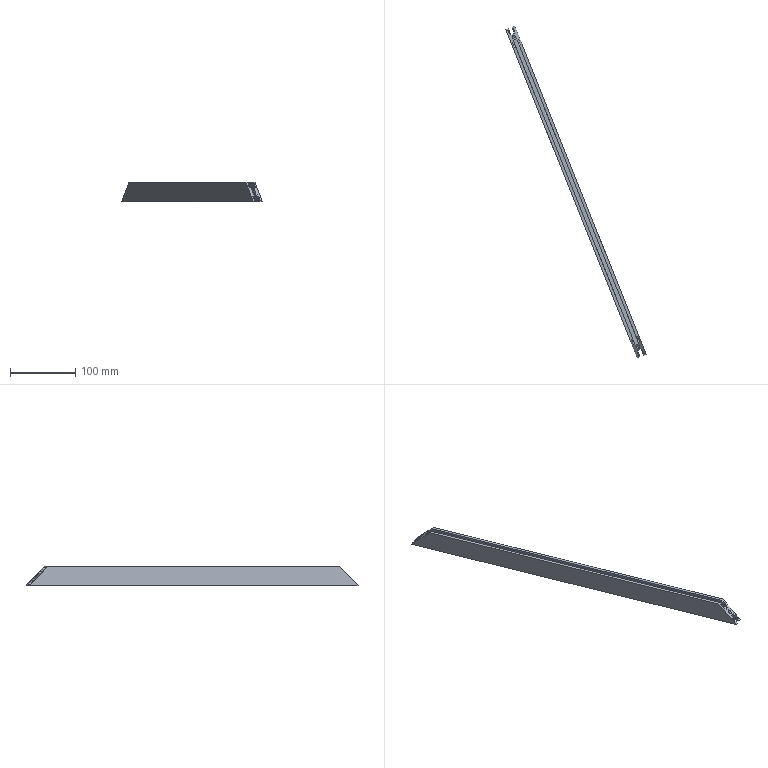Component | SolidWorks | GuardDoor-1_3015-542.5-2 | 1 solid | 32 faces | box 215.79 x 509.13 x 30 mm | volume 130208 mm3 | plane 30 | cylinder 2 | commonest cylinder face diameters 5 x2
build123d program:
from build123d import *

# Parameters (mm, degrees)
SKETCH1_R           = 2.5
BOSS_EXTRUDE1_DEPTH = 542.5
CUT_EXTRUDE1_DEPTH  = 18
CUT_EXTRUDE2_DEPTH  = 18


with BuildPart() as part:
    # Sketch1 → Boss-Extrude1 (new body)
    with BuildSketch(Plane.XY):
        Polygon((0, 0), (30, 0), (30, -4.35), (27.5, -4.35), (27.5, -2.35), (22, -2.35), (22, -4.35), (19.5, -4.35), (19.5, -10.65), (22, -10.65), (22, -12.65), (27.5, -12.65), (27.5, -10.65), (30, -10.65), (30, -15), (0, -15), (0, -10.65), (2.5, -10.65), (2.5, -12.65), (8, -12.65), (8, -10.65), (10.5, -10.65), (10.5, -4.35), (8, -4.35), (8, -2.35), (2.5, -2.35), (2.5, -4.35), (0, -4.35), align=None)
        with Locations((15, -7.5)):
            Circle(SKETCH1_R, mode=Mode.SUBTRACT)
    extrude(amount=BOSS_EXTRUDE1_DEPTH)

    # Sketch2 → Cut-Extrude1 (cut)
    with BuildSketch(Plane(origin=(0, 0, 0), x_dir=(1, 0, 0), z_dir=(0, 1, 0))):
        Polygon((0, 0), (30, -30), (30, 0), align=None)
    extrude(amount=-CUT_EXTRUDE1_DEPTH, mode=Mode.SUBTRACT)

    # Sketch3 → Cut-Extrude2 (cut)
    with BuildSketch(Plane(origin=(0, 0, 0), x_dir=(1, 0, 0), z_dir=(0, 1, 0))):
        Polygon((0, -542.5), (30, -512.5), (30, -542.5), align=None)
    extrude(amount=-CUT_EXTRUDE2_DEPTH, mode=Mode.SUBTRACT)


solid = part.part

# Placed as in the assembly
solid = solid.moved(Location((861.238, 1157.201, -420), (90, 21.845, 90)))
STEP:
#1=COLOUR_RGB('',0.7922,0.8196,0.9333);
#2=FILL_AREA_STYLE_COLOUR('',#1);
#3=FILL_AREA_STYLE('',(#2));
#4=SURFACE_STYLE_FILL_AREA(#3);
#5=SURFACE_SIDE_STYLE('',(#4));
#6=SURFACE_STYLE_USAGE(.BOTH.,#5);
#7=PRESENTATION_STYLE_ASSIGNMENT((#6));
#8=CARTESIAN_POINT('',(41.872,26.484,-15.846));
#9=VERTEX_POINT('',#8);
#10=CARTESIAN_POINT('',(41.945,26.301,-16.043));
#11=VERTEX_POINT('',#10);
#12=CARTESIAN_POINT('',(41.872,26.484,-15.846));
#13=CARTESIAN_POINT('',(42.055,26.557,-15.846));
#14=CARTESIAN_POINT('',(42.128,26.374,-16.043));
#15=CARTESIAN_POINT('',(41.945,26.301,-16.043));
#16=(BOUNDED_CURVE()B_SPLINE_CURVE(3,(#12,#13,#14,#15),.UNSPECIFIED.,.F.,.F.)B_SPLINE_CURVE_WITH_KNOTS((4,4),(-0.,3.142),.UNSPECIFIED.)CURVE()GEOMETRIC_REPRESENTATION_ITEM()RATIONAL_B_SPLINE_CURVE((1.,0.3333,0.3333,1.))REPRESENTATION_ITEM(''));
#17=EDGE_CURVE('',#9,#11,#16,.T.);
#18=ORIENTED_EDGE('',*,*,#17,.F.);
#19=CARTESIAN_POINT('',(34.437,45.029,-15.846));
#20=VERTEX_POINT('',#19);
#21=CARTESIAN_POINT('',(42.129,25.844,-15.846));
#22=DIRECTION('',(-0.3721,0.9282,0.));
#23=VECTOR('',#22,39.37);
#24=LINE('',#21,#23);
#25=EDGE_CURVE('',#9,#20,#24,.T.);
#26=ORIENTED_EDGE('',*,*,#25,.T.);
#27=CARTESIAN_POINT('',(34.364,45.212,-16.043));
#28=VERTEX_POINT('',#27);
#29=CARTESIAN_POINT('',(34.364,45.212,-16.043));
#30=CARTESIAN_POINT('',(34.547,45.285,-16.043));
#31=CARTESIAN_POINT('',(34.62,45.103,-15.846));
#32=CARTESIAN_POINT('',(34.437,45.029,-15.846));
#33=(BOUNDED_CURVE()B_SPLINE_CURVE(3,(#29,#30,#31,#32),.UNSPECIFIED.,.F.,.T.)B_SPLINE_CURVE_WITH_KNOTS((4,4),(-0.,3.142),.UNSPECIFIED.)CURVE()GEOMETRIC_REPRESENTATION_ITEM()RATIONAL_B_SPLINE_CURVE((1.,0.3333,0.3333,1.))REPRESENTATION_ITEM(''));
#34=EDGE_CURVE('',#28,#20,#33,.T.);
#35=ORIENTED_EDGE('',*,*,#34,.F.);
#36=CARTESIAN_POINT('',(42.129,25.844,-16.043));
#37=DIRECTION('',(-0.3721,0.9282,0.));
#38=VECTOR('',#37,39.37);
#39=LINE('',#36,#38);
#40=EDGE_CURVE('',#11,#28,#39,.T.);
#41=ORIENTED_EDGE('',*,*,#40,.F.);
#42=EDGE_LOOP('',(#18,#26,#35,#41));
#43=FACE_OUTER_BOUND('',#42,.T.);
#44=CARTESIAN_POINT('',(42.129,25.844,-15.945));
#45=DIRECTION('',(-0.3721,0.9282,0.));
#46=DIRECTION('',(0.,0.,-1.));
#47=AXIS2_PLACEMENT_3D('',#44,#45,#46);
#48=CYLINDRICAL_SURFACE('',#47,0.09843);
#49=ADVANCED_FACE('',(#43),#48,.F.);
#50=CARTESIAN_POINT('',(33.907,45.559,-16.535));
#51=VERTEX_POINT('',#50);
#52=CARTESIAN_POINT('',(34.066,45.623,-16.535));
#53=VERTEX_POINT('',#52);
#54=CARTESIAN_POINT('',(33.907,45.559,-16.535));
#55=DIRECTION('',(0.9282,0.3721,-0.));
#56=VECTOR('',#55,39.37);
#57=LINE('',#54,#56);
#58=EDGE_CURVE('',#51,#53,#57,.T.);
#59=ORIENTED_EDGE('',*,*,#58,.T.);
#60=CARTESIAN_POINT('',(42.013,25.798,-16.535));
#61=VERTEX_POINT('',#60);
#62=CARTESIAN_POINT('',(42.013,25.798,-16.535));
#63=DIRECTION('',(-0.3721,0.9282,0.));
#64=VECTOR('',#63,39.37);
#65=LINE('',#62,#64);
#66=EDGE_CURVE('',#61,#53,#65,.T.);
#67=ORIENTED_EDGE('',*,*,#66,.F.);
#68=CARTESIAN_POINT('',(41.854,25.735,-16.535));
#69=VERTEX_POINT('',#68);
#70=CARTESIAN_POINT('',(41.854,25.735,-16.535));
#71=DIRECTION('',(0.9282,0.3721,-0.));
#72=VECTOR('',#71,39.37);
#73=LINE('',#70,#72);
#74=EDGE_CURVE('',#69,#61,#73,.T.);
#75=ORIENTED_EDGE('',*,*,#74,.F.);
#76=CARTESIAN_POINT('',(41.854,25.735,-16.535));
#77=DIRECTION('',(-0.3721,0.9282,0.));
#78=VECTOR('',#77,39.37);
#79=LINE('',#76,#78);
#80=EDGE_CURVE('',#69,#51,#79,.T.);
#81=ORIENTED_EDGE('',*,*,#80,.T.);
#82=EDGE_LOOP('',(#59,#67,#75,#81));
#83=FACE_OUTER_BOUND('',#82,.T.);
#84=CARTESIAN_POINT('',(41.854,25.735,-16.535));
#85=DIRECTION('',(0.,-0.,1.));
#86=DIRECTION('',(-0.9282,-0.3721,0.));
#87=AXIS2_PLACEMENT_3D('',#84,#85,#86);
#88=PLANE('',#87);
#89=ADVANCED_FACE('',(#83),#88,.F.);
#90=CARTESIAN_POINT('',(41.977,25.89,-16.437));
#91=VERTEX_POINT('',#90);
#92=CARTESIAN_POINT('',(34.103,45.531,-16.437));
#93=VERTEX_POINT('',#92);
#94=CARTESIAN_POINT('',(42.013,25.798,-16.437));
#95=DIRECTION('',(-0.3721,0.9282,0.));
#96=VECTOR('',#95,39.37);
#97=LINE('',#94,#96);
#98=EDGE_CURVE('',#91,#93,#97,.T.);
#99=ORIENTED_EDGE('',*,*,#98,.F.);
#100=CARTESIAN_POINT('',(42.013,25.798,-16.535));
#101=DIRECTION('',(0.2631,-0.6563,-0.7071));
#102=VECTOR('',#101,39.37);
#103=LINE('',#100,#102);
#104=EDGE_CURVE('',#91,#61,#103,.T.);
#105=ORIENTED_EDGE('',*,*,#104,.T.);
#106=ORIENTED_EDGE('',*,*,#66,.T.);
#107=CARTESIAN_POINT('',(38.04,35.711,-5.856));
#108=DIRECTION('',(0.2631,-0.6563,0.7071));
#109=VECTOR('',#108,39.37);
#110=LINE('',#107,#109);
#111=EDGE_CURVE('',#53,#93,#110,.T.);
#112=ORIENTED_EDGE('',*,*,#111,.T.);
#113=EDGE_LOOP('',(#99,#105,#106,#112));
#114=FACE_OUTER_BOUND('',#113,.T.);
#115=CARTESIAN_POINT('',(42.013,25.798,-16.535));
#116=DIRECTION('',(-0.9282,-0.3721,0.));
#117=DIRECTION('',(0.3721,-0.9282,-0.));
#118=AXIS2_PLACEMENT_3D('',#115,#116,#117);
#119=PLANE('',#118);
#120=ADVANCED_FACE('',(#114),#119,.F.);
#121=CARTESIAN_POINT('',(41.904,25.86,-16.437));
#122=VERTEX_POINT('',#121);
#123=CARTESIAN_POINT('',(34.029,45.502,-16.437));
#124=VERTEX_POINT('',#123);
#125=CARTESIAN_POINT('',(41.94,25.769,-16.437));
#126=DIRECTION('',(-0.3721,0.9282,0.));
#127=VECTOR('',#126,39.37);
#128=LINE('',#125,#127);
#129=EDGE_CURVE('',#122,#124,#128,.T.);
#130=ORIENTED_EDGE('',*,*,#129,.F.);
#131=CARTESIAN_POINT('',(41.977,25.89,-16.437));
#132=DIRECTION('',(0.9282,0.3721,-0.));
#133=VECTOR('',#132,39.37);
#134=LINE('',#131,#133);
#135=EDGE_CURVE('',#122,#91,#134,.T.);
#136=ORIENTED_EDGE('',*,*,#135,.T.);
#137=ORIENTED_EDGE('',*,*,#98,.T.);
#138=CARTESIAN_POINT('',(34.103,45.531,-16.437));
#139=DIRECTION('',(-0.9282,-0.3721,0.));
#140=VECTOR('',#139,39.37);
#141=LINE('',#138,#140);
#142=EDGE_CURVE('',#93,#124,#141,.T.);
#143=ORIENTED_EDGE('',*,*,#142,.T.);
#144=EDGE_LOOP('',(#130,#136,#137,#143));
#145=FACE_OUTER_BOUND('',#144,.T.);
#146=CARTESIAN_POINT('',(42.013,25.798,-16.437));
#147=DIRECTION('',(-0.,0.,-1.));
#148=DIRECTION('',(0.3721,-0.9282,-0.));
#149=AXIS2_PLACEMENT_3D('',#146,#147,#148);
#150=PLANE('',#149);
#151=ADVANCED_FACE('',(#145),#150,.F.);
#152=CARTESIAN_POINT('',(41.823,26.061,-16.22));
#153=VERTEX_POINT('',#152);
#154=CARTESIAN_POINT('',(34.11,45.301,-16.22));
#155=VERTEX_POINT('',#154);
#156=CARTESIAN_POINT('',(41.94,25.769,-16.22));
#157=DIRECTION('',(-0.3721,0.9282,0.));
#158=VECTOR('',#157,39.37);
#159=LINE('',#156,#158);
#160=EDGE_CURVE('',#153,#155,#159,.T.);
#161=ORIENTED_EDGE('',*,*,#160,.F.);
#162=CARTESIAN_POINT('',(41.922,25.815,-16.486));
#163=DIRECTION('',(0.2631,-0.6563,-0.7071));
#164=VECTOR('',#163,39.37);
#165=LINE('',#162,#164);
#166=EDGE_CURVE('',#153,#122,#165,.T.);
#167=ORIENTED_EDGE('',*,*,#166,.T.);
#168=ORIENTED_EDGE('',*,*,#129,.T.);
#169=CARTESIAN_POINT('',(37.985,35.636,-5.807));
#170=DIRECTION('',(0.2631,-0.6563,0.7071));
#171=VECTOR('',#170,39.37);
#172=LINE('',#169,#171);
#173=EDGE_CURVE('',#124,#155,#172,.T.);
#174=ORIENTED_EDGE('',*,*,#173,.T.);
#175=EDGE_LOOP('',(#161,#167,#168,#174));
#176=FACE_OUTER_BOUND('',#175,.T.);
#177=CARTESIAN_POINT('',(41.94,25.769,-16.437));
#178=DIRECTION('',(-0.9282,-0.3721,0.));
#179=DIRECTION('',(0.3721,-0.9282,-0.));
#180=AXIS2_PLACEMENT_3D('',#177,#178,#179);
#181=PLANE('',#180);
#182=ADVANCED_FACE('',(#176),#181,.F.);
#183=CARTESIAN_POINT('',(41.896,26.091,-16.22));
#184=VERTEX_POINT('',#183);
#185=CARTESIAN_POINT('',(34.183,45.33,-16.22));
#186=VERTEX_POINT('',#185);
#187=CARTESIAN_POINT('',(42.013,25.798,-16.22));
#188=DIRECTION('',(-0.3721,0.9282,0.));
#189=VECTOR('',#188,39.37);
#190=LINE('',#187,#189);
#191=EDGE_CURVE('',#184,#186,#190,.T.);
#192=ORIENTED_EDGE('',*,*,#191,.F.);
#193=CARTESIAN_POINT('',(41.823,26.061,-16.22));
#194=DIRECTION('',(-0.9282,-0.3721,0.));
#195=VECTOR('',#194,39.37);
#196=LINE('',#193,#195);
#197=EDGE_CURVE('',#184,#153,#196,.T.);
#198=ORIENTED_EDGE('',*,*,#197,.T.);
#199=ORIENTED_EDGE('',*,*,#160,.T.);
#200=CARTESIAN_POINT('',(34.11,45.301,-16.22));
#201=DIRECTION('',(0.9282,0.3721,-0.));
#202=VECTOR('',#201,39.37);
#203=LINE('',#200,#202);
#204=EDGE_CURVE('',#155,#186,#203,.T.);
#205=ORIENTED_EDGE('',*,*,#204,.T.);
#206=EDGE_LOOP('',(#192,#198,#199,#205));
#207=FACE_OUTER_BOUND('',#206,.T.);
#208=CARTESIAN_POINT('',(41.94,25.769,-16.22));
#209=DIRECTION('',(0.,-0.,1.));
#210=DIRECTION('',(-0.3721,0.9282,0.));
#211=AXIS2_PLACEMENT_3D('',#208,#209,#210);
#212=PLANE('',#211);
#213=ADVANCED_FACE('',(#207),#212,.F.);
#214=CARTESIAN_POINT('',(41.86,26.182,-16.122));
#215=VERTEX_POINT('',#214);
#216=CARTESIAN_POINT('',(34.22,45.239,-16.122));
#217=VERTEX_POINT('',#216);
#218=CARTESIAN_POINT('',(42.013,25.798,-16.122));
#219=DIRECTION('',(-0.3721,0.9282,0.));
#220=VECTOR('',#219,39.37);
#221=LINE('',#218,#220);
#222=EDGE_CURVE('',#215,#217,#221,.T.);
#223=ORIENTED_EDGE('',*,*,#222,.F.);
#224=CARTESIAN_POINT('',(41.955,25.944,-16.378));
#225=DIRECTION('',(0.2631,-0.6563,-0.7071));
#226=VECTOR('',#225,39.37);
#227=LINE('',#224,#226);
#228=EDGE_CURVE('',#215,#184,#227,.T.);
#229=ORIENTED_EDGE('',*,*,#228,.T.);
#230=ORIENTED_EDGE('',*,*,#191,.T.);
#231=CARTESIAN_POINT('',(38.098,35.564,-5.699));
#232=DIRECTION('',(0.2631,-0.6563,0.7071));
#233=VECTOR('',#232,39.37);
#234=LINE('',#231,#233);
#235=EDGE_CURVE('',#186,#217,#234,.T.);
#236=ORIENTED_EDGE('',*,*,#235,.T.);
#237=EDGE_LOOP('',(#223,#229,#230,#236));
#238=FACE_OUTER_BOUND('',#237,.T.);
#239=CARTESIAN_POINT('',(42.013,25.798,-16.22));
#240=DIRECTION('',(-0.9282,-0.3721,0.));
#241=DIRECTION('',(0.3721,-0.9282,-0.));
#242=AXIS2_PLACEMENT_3D('',#239,#240,#241);
#243=PLANE('',#242);
#244=ADVANCED_FACE('',(#238),#243,.F.);
#245=CARTESIAN_POINT('',(42.09,26.274,-16.122));
#246=VERTEX_POINT('',#245);
#247=CARTESIAN_POINT('',(34.45,45.331,-16.122));
#248=VERTEX_POINT('',#247);
#249=CARTESIAN_POINT('',(42.244,25.891,-16.122));
#250=DIRECTION('',(-0.3721,0.9282,0.));
#251=VECTOR('',#250,39.37);
#252=LINE('',#249,#251);
#253=EDGE_CURVE('',#246,#248,#252,.T.);
#254=ORIENTED_EDGE('',*,*,#253,.F.);
#255=CARTESIAN_POINT('',(41.86,26.182,-16.122));
#256=DIRECTION('',(-0.9282,-0.3721,0.));
#257=VECTOR('',#256,39.37);
#258=LINE('',#255,#257);
#259=EDGE_CURVE('',#246,#215,#258,.T.);
#260=ORIENTED_EDGE('',*,*,#259,.T.);
#261=ORIENTED_EDGE('',*,*,#222,.T.);
#262=CARTESIAN_POINT('',(34.22,45.239,-16.122));
#263=DIRECTION('',(0.9282,0.3721,-0.));
#264=VECTOR('',#263,39.37);
#265=LINE('',#262,#264);
#266=EDGE_CURVE('',#217,#248,#265,.T.);
#267=ORIENTED_EDGE('',*,*,#266,.T.);
#268=EDGE_LOOP('',(#254,#260,#261,#267));
#269=FACE_OUTER_BOUND('',#268,.T.);
#270=CARTESIAN_POINT('',(42.013,25.798,-16.122));
#271=DIRECTION('',(0.,-0.,1.));
#272=DIRECTION('',(-0.9282,-0.3721,0.));
#273=AXIS2_PLACEMENT_3D('',#270,#271,#272);
#274=PLANE('',#273);
#275=ADVANCED_FACE('',(#269),#274,.F.);
#276=CARTESIAN_POINT('',(42.126,26.183,-16.22));
#277=VERTEX_POINT('',#276);
#278=CARTESIAN_POINT('',(34.413,45.423,-16.22));
#279=VERTEX_POINT('',#278);
#280=CARTESIAN_POINT('',(42.244,25.891,-16.22));
#281=DIRECTION('',(-0.3721,0.9282,0.));
#282=VECTOR('',#281,39.37);
#283=LINE('',#280,#282);
#284=EDGE_CURVE('',#277,#279,#283,.T.);
#285=ORIENTED_EDGE('',*,*,#284,.F.);
#286=CARTESIAN_POINT('',(42.185,26.037,-16.378));
#287=DIRECTION('',(-0.2631,0.6563,0.7071));
#288=VECTOR('',#287,39.37);
#289=LINE('',#286,#288);
#290=EDGE_CURVE('',#277,#246,#289,.T.);
#291=ORIENTED_EDGE('',*,*,#290,.T.);
#292=ORIENTED_EDGE('',*,*,#253,.T.);
#293=CARTESIAN_POINT('',(38.329,35.657,-5.699));
#294=DIRECTION('',(-0.2631,0.6563,-0.7071));
#295=VECTOR('',#294,39.37);
#296=LINE('',#293,#295);
#297=EDGE_CURVE('',#248,#279,#296,.T.);
#298=ORIENTED_EDGE('',*,*,#297,.T.);
#299=EDGE_LOOP('',(#285,#291,#292,#298));
#300=FACE_OUTER_BOUND('',#299,.T.);
#301=CARTESIAN_POINT('',(42.244,25.891,-16.22));
#302=DIRECTION('',(0.9282,0.3721,-0.));
#303=DIRECTION('',(-0.3721,0.9282,0.));
#304=AXIS2_PLACEMENT_3D('',#301,#302,#303);
#305=PLANE('',#304);
#306=ADVANCED_FACE('',(#300),#305,.F.);
#307=CARTESIAN_POINT('',(42.2,26.212,-16.22));
#308=VERTEX_POINT('',#307);
#309=CARTESIAN_POINT('',(34.486,45.452,-16.22));
#310=VERTEX_POINT('',#309);
#311=CARTESIAN_POINT('',(42.317,25.92,-16.22));
#312=DIRECTION('',(-0.3721,0.9282,0.));
#313=VECTOR('',#312,39.37);
#314=LINE('',#311,#313);
#315=EDGE_CURVE('',#308,#310,#314,.T.);
#316=ORIENTED_EDGE('',*,*,#315,.F.);
#317=CARTESIAN_POINT('',(42.2,26.212,-16.22));
#318=DIRECTION('',(-0.9282,-0.3721,0.));
#319=VECTOR('',#318,39.37);
#320=LINE('',#317,#319);
#321=EDGE_CURVE('',#308,#277,#320,.T.);
#322=ORIENTED_EDGE('',*,*,#321,.T.);
#323=ORIENTED_EDGE('',*,*,#284,.T.);
#324=CARTESIAN_POINT('',(34.486,45.452,-16.22));
#325=DIRECTION('',(0.9282,0.3721,-0.));
#326=VECTOR('',#325,39.37);
#327=LINE('',#324,#326);
#328=EDGE_CURVE('',#279,#310,#327,.T.);
#329=ORIENTED_EDGE('',*,*,#328,.T.);
#330=EDGE_LOOP('',(#316,#322,#323,#329));
#331=FACE_OUTER_BOUND('',#330,.T.);
#332=CARTESIAN_POINT('',(42.317,25.92,-16.22));
#333=DIRECTION('',(0.,-0.,1.));
#334=DIRECTION('',(-0.3721,0.9282,0.));
#335=AXIS2_PLACEMENT_3D('',#332,#333,#334);
#336=PLANE('',#335);
#337=ADVANCED_FACE('',(#331),#336,.F.);
#338=CARTESIAN_POINT('',(42.28,26.011,-16.437));
#339=VERTEX_POINT('',#338);
#340=CARTESIAN_POINT('',(34.406,45.653,-16.437));
#341=VERTEX_POINT('',#340);
#342=CARTESIAN_POINT('',(42.317,25.92,-16.437));
#343=DIRECTION('',(-0.3721,0.9282,0.));
#344=VECTOR('',#343,39.37);
#345=LINE('',#342,#344);
#346=EDGE_CURVE('',#339,#341,#345,.T.);
#347=ORIENTED_EDGE('',*,*,#346,.F.);
#348=CARTESIAN_POINT('',(42.298,25.966,-16.486));
#349=DIRECTION('',(-0.2631,0.6563,0.7071));
#350=VECTOR('',#349,39.37);
#351=LINE('',#348,#350);
#352=EDGE_CURVE('',#339,#308,#351,.T.);
#353=ORIENTED_EDGE('',*,*,#352,.T.);
#354=ORIENTED_EDGE('',*,*,#315,.T.);
#355=CARTESIAN_POINT('',(38.361,35.786,-5.807));
#356=DIRECTION('',(-0.2631,0.6563,-0.7071));
#357=VECTOR('',#356,39.37);
#358=LINE('',#355,#357);
#359=EDGE_CURVE('',#310,#341,#358,.T.);
#360=ORIENTED_EDGE('',*,*,#359,.T.);
#361=EDGE_LOOP('',(#347,#353,#354,#360));
#362=FACE_OUTER_BOUND('',#361,.T.);
#363=CARTESIAN_POINT('',(42.317,25.92,-16.437));
#364=DIRECTION('',(0.9282,0.3721,-0.));
#365=DIRECTION('',(-0.3721,0.9282,0.));
#366=AXIS2_PLACEMENT_3D('',#363,#364,#365);
#367=PLANE('',#366);
#368=ADVANCED_FACE('',(#362),#367,.F.);
#369=CARTESIAN_POINT('',(42.207,25.982,-16.437));
#370=VERTEX_POINT('',#369);
#371=CARTESIAN_POINT('',(34.333,45.624,-16.437));
#372=VERTEX_POINT('',#371);
#373=CARTESIAN_POINT('',(42.244,25.891,-16.437));
#374=DIRECTION('',(-0.3721,0.9282,0.));
#375=VECTOR('',#374,39.37);
#376=LINE('',#373,#375);
#377=EDGE_CURVE('',#370,#372,#376,.T.);
#378=ORIENTED_EDGE('',*,*,#377,.F.);
#379=CARTESIAN_POINT('',(42.207,25.982,-16.437));
#380=DIRECTION('',(0.9282,0.3721,-0.));
#381=VECTOR('',#380,39.37);
#382=LINE('',#379,#381);
#383=EDGE_CURVE('',#370,#339,#382,.T.);
#384=ORIENTED_EDGE('',*,*,#383,.T.);
#385=ORIENTED_EDGE('',*,*,#346,.T.);
#386=CARTESIAN_POINT('',(34.333,45.624,-16.437));
#387=DIRECTION('',(-0.9282,-0.3721,0.));
#388=VECTOR('',#387,39.37);
#389=LINE('',#386,#388);
#390=EDGE_CURVE('',#341,#372,#389,.T.);
#391=ORIENTED_EDGE('',*,*,#390,.T.);
#392=EDGE_LOOP('',(#378,#384,#385,#391));
#393=FACE_OUTER_BOUND('',#392,.T.);
#394=CARTESIAN_POINT('',(42.244,25.891,-16.437));
#395=DIRECTION('',(-0.,0.,-1.));
#396=DIRECTION('',(0.3721,-0.9282,-0.));
#397=AXIS2_PLACEMENT_3D('',#394,#395,#396);
#398=PLANE('',#397);
#399=ADVANCED_FACE('',(#393),#398,.F.);
#400=CARTESIAN_POINT('',(42.244,25.891,-16.535));
#401=VERTEX_POINT('',#400);
#402=CARTESIAN_POINT('',(34.296,45.715,-16.535));
#403=VERTEX_POINT('',#402);
#404=CARTESIAN_POINT('',(42.244,25.891,-16.535));
#405=DIRECTION('',(-0.3721,0.9282,0.));
#406=VECTOR('',#405,39.37);
#407=LINE('',#404,#406);
#408=EDGE_CURVE('',#401,#403,#407,.T.);
#409=ORIENTED_EDGE('',*,*,#408,.F.);
#410=CARTESIAN_POINT('',(42.244,25.891,-16.535));
#411=DIRECTION('',(-0.2631,0.6563,0.7071));
#412=VECTOR('',#411,39.37);
#413=LINE('',#410,#412);
#414=EDGE_CURVE('',#401,#370,#413,.T.);
#415=ORIENTED_EDGE('',*,*,#414,.T.);
#416=ORIENTED_EDGE('',*,*,#377,.T.);
#417=CARTESIAN_POINT('',(38.27,35.803,-5.856));
#418=DIRECTION('',(-0.2631,0.6563,-0.7071));
#419=VECTOR('',#418,39.37);
#420=LINE('',#417,#419);
#421=EDGE_CURVE('',#372,#403,#420,.T.);
#422=ORIENTED_EDGE('',*,*,#421,.T.);
#423=EDGE_LOOP('',(#409,#415,#416,#422));
#424=FACE_OUTER_BOUND('',#423,.T.);
#425=CARTESIAN_POINT('',(42.244,25.891,-16.535));
#426=DIRECTION('',(0.9282,0.3721,-0.));
#427=DIRECTION('',(-0.3721,0.9282,0.));
#428=AXIS2_PLACEMENT_3D('',#425,#426,#427);
#429=PLANE('',#428);
#430=ADVANCED_FACE('',(#424),#429,.F.);
#431=CARTESIAN_POINT('',(34.455,45.779,-16.535));
#432=VERTEX_POINT('',#431);
#433=CARTESIAN_POINT('',(34.296,45.715,-16.535));
#434=DIRECTION('',(0.9282,0.3721,0.));
#435=VECTOR('',#434,39.37);
#436=LINE('',#433,#435);
#437=EDGE_CURVE('',#403,#432,#436,.T.);
#438=ORIENTED_EDGE('',*,*,#437,.T.);
#439=CARTESIAN_POINT('',(42.403,25.954,-16.535));
#440=VERTEX_POINT('',#439);
#441=CARTESIAN_POINT('',(42.403,25.954,-16.535));
#442=DIRECTION('',(-0.3721,0.9282,0.));
#443=VECTOR('',#442,39.37);
#444=LINE('',#441,#443);
#445=EDGE_CURVE('',#440,#432,#444,.T.);
#446=ORIENTED_EDGE('',*,*,#445,.F.);
#447=CARTESIAN_POINT('',(42.244,25.891,-16.535));
#448=DIRECTION('',(0.9282,0.3721,0.));
#449=VECTOR('',#448,39.37);
#450=LINE('',#447,#449);
#451=EDGE_CURVE('',#401,#440,#450,.T.);
#452=ORIENTED_EDGE('',*,*,#451,.F.);
#453=ORIENTED_EDGE('',*,*,#408,.T.);
#454=EDGE_LOOP('',(#438,#446,#452,#453));
#455=FACE_OUTER_BOUND('',#454,.T.);
#456=CARTESIAN_POINT('',(42.244,25.891,-16.535));
#457=DIRECTION('',(0.,-0.,1.));
#458=DIRECTION('',(-0.9282,-0.3721,-0.));
#459=AXIS2_PLACEMENT_3D('',#456,#457,#458);
#460=PLANE('',#459);
#461=ADVANCED_FACE('',(#455),#460,.F.);
#462=CARTESIAN_POINT('',(41.963,27.051,-15.354));
#463=VERTEX_POINT('',#462);
#464=CARTESIAN_POINT('',(34.895,44.683,-15.354));
#465=VERTEX_POINT('',#464);
#466=CARTESIAN_POINT('',(42.403,25.954,-15.354));
#467=DIRECTION('',(-0.3721,0.9282,0.));
#468=VECTOR('',#467,39.37);
#469=LINE('',#466,#468);
#470=EDGE_CURVE('',#463,#465,#469,.T.);
#471=ORIENTED_EDGE('',*,*,#470,.F.);
#472=CARTESIAN_POINT('',(42.403,25.954,-16.535));
#473=DIRECTION('',(0.2631,-0.6563,-0.7071));
#474=VECTOR('',#473,39.37);
#475=LINE('',#472,#474);
#476=EDGE_CURVE('',#463,#440,#475,.T.);
#477=ORIENTED_EDGE('',*,*,#476,.T.);
#478=ORIENTED_EDGE('',*,*,#445,.T.);
#479=CARTESIAN_POINT('',(38.429,35.867,-5.856));
#480=DIRECTION('',(0.2631,-0.6563,0.7071));
#481=VECTOR('',#480,39.37);
#482=LINE('',#479,#481);
#483=EDGE_CURVE('',#432,#465,#482,.T.);
#484=ORIENTED_EDGE('',*,*,#483,.T.);
#485=EDGE_LOOP('',(#471,#477,#478,#484));
#486=FACE_OUTER_BOUND('',#485,.T.);
#487=CARTESIAN_POINT('',(42.403,25.954,-16.535));
#488=DIRECTION('',(-0.9282,-0.3721,0.));
#489=DIRECTION('',(0.3721,-0.9282,-0.));
#490=AXIS2_PLACEMENT_3D('',#487,#488,#489);
#491=PLANE('',#490);
#492=ADVANCED_FACE('',(#486),#491,.F.);
#493=CARTESIAN_POINT('',(41.804,26.987,-15.354));
#494=VERTEX_POINT('',#493);
#495=CARTESIAN_POINT('',(34.736,44.619,-15.354));
#496=VERTEX_POINT('',#495);
#497=CARTESIAN_POINT('',(42.244,25.891,-15.354));
#498=DIRECTION('',(-0.3721,0.9282,0.));
#499=VECTOR('',#498,39.37);
#500=LINE('',#497,#499);
#501=EDGE_CURVE('',#494,#496,#500,.T.);
#502=ORIENTED_EDGE('',*,*,#501,.F.);
#503=CARTESIAN_POINT('',(42.073,27.095,-15.354));
#504=DIRECTION('',(-0.9282,-0.3721,0.));
#505=VECTOR('',#504,39.37);
#506=LINE('',#503,#505);
#507=EDGE_CURVE('',#463,#494,#506,.T.);
#508=ORIENTED_EDGE('',*,*,#507,.F.);
#509=ORIENTED_EDGE('',*,*,#470,.T.);
#510=CARTESIAN_POINT('',(35.004,44.727,-15.354));
#511=DIRECTION('',(-0.9282,-0.3721,0.));
#512=VECTOR('',#511,39.37);
#513=LINE('',#510,#512);
#514=EDGE_CURVE('',#465,#496,#513,.T.);
#515=ORIENTED_EDGE('',*,*,#514,.T.);
#516=EDGE_LOOP('',(#502,#508,#509,#515));
#517=FACE_OUTER_BOUND('',#516,.T.);
#518=CARTESIAN_POINT('',(42.244,25.891,-15.354));
#519=DIRECTION('',(0.,0.,-1.));
#520=DIRECTION('',(0.9282,0.3721,0.));
#521=AXIS2_PLACEMENT_3D('',#518,#519,#520);
#522=PLANE('',#521);
#523=ADVANCED_FACE('',(#517),#522,.F.);
#524=CARTESIAN_POINT('',(41.841,26.895,-15.453));
#525=VERTEX_POINT('',#524);
#526=CARTESIAN_POINT('',(34.699,44.71,-15.453));
#527=VERTEX_POINT('',#526);
#528=CARTESIAN_POINT('',(42.244,25.891,-15.453));
#529=DIRECTION('',(-0.3721,0.9282,0.));
#530=VECTOR('',#529,39.37);
#531=LINE('',#528,#530);
#532=EDGE_CURVE('',#525,#527,#531,.T.);
#533=ORIENTED_EDGE('',*,*,#532,.F.);
#534=CARTESIAN_POINT('',(42.024,26.439,-15.945));
#535=DIRECTION('',(-0.2631,0.6563,0.7071));
#536=VECTOR('',#535,39.37);
#537=LINE('',#534,#536);
#538=EDGE_CURVE('',#525,#494,#537,.T.);
#539=ORIENTED_EDGE('',*,*,#538,.T.);
#540=ORIENTED_EDGE('',*,*,#501,.T.);
#541=CARTESIAN_POINT('',(38.49,35.255,-5.266));
#542=DIRECTION('',(-0.2631,0.6563,-0.7071));
#543=VECTOR('',#542,39.37);
#544=LINE('',#541,#543);
#545=EDGE_CURVE('',#496,#527,#544,.T.);
#546=ORIENTED_EDGE('',*,*,#545,.T.);
#547=EDGE_LOOP('',(#533,#539,#540,#546));
#548=FACE_OUTER_BOUND('',#547,.T.);
#549=CARTESIAN_POINT('',(42.244,25.891,-15.354));
#550=DIRECTION('',(0.9282,0.3721,-0.));
#551=DIRECTION('',(-0.3721,0.9282,0.));
#552=AXIS2_PLACEMENT_3D('',#549,#550,#551);
#553=PLANE('',#552);
#554=ADVANCED_FACE('',(#548),#553,.F.);
#555=CARTESIAN_POINT('',(41.914,26.925,-15.453));
#556=VERTEX_POINT('',#555);
#557=CARTESIAN_POINT('',(34.772,44.739,-15.453));
#558=VERTEX_POINT('',#557);
#559=CARTESIAN_POINT('',(42.317,25.92,-15.453));
#560=DIRECTION('',(-0.3721,0.9282,0.));
#561=VECTOR('',#560,39.37);
#562=LINE('',#559,#561);
#563=EDGE_CURVE('',#556,#558,#562,.T.);
#564=ORIENTED_EDGE('',*,*,#563,.F.);
#565=CARTESIAN_POINT('',(41.841,26.895,-15.453));
#566=DIRECTION('',(-0.9282,-0.3721,0.));
#567=VECTOR('',#566,39.37);
#568=LINE('',#565,#567);
#569=EDGE_CURVE('',#556,#525,#568,.T.);
#570=ORIENTED_EDGE('',*,*,#569,.T.);
#571=ORIENTED_EDGE('',*,*,#532,.T.);
#572=CARTESIAN_POINT('',(34.699,44.71,-15.453));
#573=DIRECTION('',(0.9282,0.3721,-0.));
#574=VECTOR('',#573,39.37);
#575=LINE('',#572,#574);
#576=EDGE_CURVE('',#527,#558,#575,.T.);
#577=ORIENTED_EDGE('',*,*,#576,.T.);
#578=EDGE_LOOP('',(#564,#570,#571,#577));
#579=FACE_OUTER_BOUND('',#578,.T.);
#580=CARTESIAN_POINT('',(42.244,25.891,-15.453));
#581=DIRECTION('',(0.,-0.,1.));
#582=DIRECTION('',(-0.3721,0.9282,0.));
#583=AXIS2_PLACEMENT_3D('',#580,#581,#582);
#584=PLANE('',#583);
#585=ADVANCED_FACE('',(#579),#584,.F.);
#586=CARTESIAN_POINT('',(41.994,26.724,-15.669));
#587=VERTEX_POINT('',#586);
#588=CARTESIAN_POINT('',(34.692,44.94,-15.669));
#589=VERTEX_POINT('',#588);
#590=CARTESIAN_POINT('',(42.317,25.92,-15.669));
#591=DIRECTION('',(-0.3721,0.9282,0.));
#592=VECTOR('',#591,39.37);
#593=LINE('',#590,#592);
#594=EDGE_CURVE('',#587,#589,#593,.T.);
#595=ORIENTED_EDGE('',*,*,#594,.F.);
#596=CARTESIAN_POINT('',(42.115,26.422,-15.994));
#597=DIRECTION('',(-0.2631,0.6563,0.7071));
#598=VECTOR('',#597,39.37);
#599=LINE('',#596,#598);
#600=EDGE_CURVE('',#587,#556,#599,.T.);
#601=ORIENTED_EDGE('',*,*,#600,.T.);
#602=ORIENTED_EDGE('',*,*,#563,.T.);
#603=CARTESIAN_POINT('',(38.544,35.33,-5.315));
#604=DIRECTION('',(-0.2631,0.6563,-0.7071));
#605=VECTOR('',#604,39.37);
#606=LINE('',#603,#605);
#607=EDGE_CURVE('',#558,#589,#606,.T.);
#608=ORIENTED_EDGE('',*,*,#607,.T.);
#609=EDGE_LOOP('',(#595,#601,#602,#608));
#610=FACE_OUTER_BOUND('',#609,.T.);
#611=CARTESIAN_POINT('',(42.317,25.92,-15.453));
#612=DIRECTION('',(0.9282,0.3721,-0.));
#613=DIRECTION('',(-0.3721,0.9282,0.));
#614=AXIS2_PLACEMENT_3D('',#611,#612,#613);
#615=PLANE('',#614);
#616=ADVANCED_FACE('',(#610),#615,.F.);
#617=CARTESIAN_POINT('',(41.921,26.695,-15.669));
#618=VERTEX_POINT('',#617);
#619=CARTESIAN_POINT('',(34.618,44.911,-15.669));
#620=VERTEX_POINT('',#619);
#621=CARTESIAN_POINT('',(42.244,25.891,-15.669));
#622=DIRECTION('',(-0.3721,0.9282,0.));
#623=VECTOR('',#622,39.37);
#624=LINE('',#621,#623);
#625=EDGE_CURVE('',#618,#620,#624,.T.);
#626=ORIENTED_EDGE('',*,*,#625,.F.);
#627=CARTESIAN_POINT('',(41.994,26.724,-15.669));
#628=DIRECTION('',(0.9282,0.3721,-0.));
#629=VECTOR('',#628,39.37);
#630=LINE('',#627,#629);
#631=EDGE_CURVE('',#618,#587,#630,.T.);
#632=ORIENTED_EDGE('',*,*,#631,.T.);
#633=ORIENTED_EDGE('',*,*,#594,.T.);
#634=CARTESIAN_POINT('',(34.692,44.94,-15.669));
#635=DIRECTION('',(-0.9282,-0.3721,0.));
#636=VECTOR('',#635,39.37);
#637=LINE('',#634,#636);
#638=EDGE_CURVE('',#589,#620,#637,.T.);
#639=ORIENTED_EDGE('',*,*,#638,.T.);
#640=EDGE_LOOP('',(#626,#632,#633,#639));
#641=FACE_OUTER_BOUND('',#640,.T.);
#642=CARTESIAN_POINT('',(42.317,25.92,-15.669));
#643=DIRECTION('',(-0.,0.,-1.));
#644=DIRECTION('',(0.3721,-0.9282,-0.));
#645=AXIS2_PLACEMENT_3D('',#642,#643,#644);
#646=PLANE('',#645);
#647=ADVANCED_FACE('',(#641),#646,.F.);
#648=CARTESIAN_POINT('',(41.958,26.603,-15.768));
#649=VERTEX_POINT('',#648);
#650=CARTESIAN_POINT('',(34.582,45.003,-15.768));
#651=VERTEX_POINT('',#650);
#652=CARTESIAN_POINT('',(42.244,25.891,-15.768));
#653=DIRECTION('',(-0.3721,0.9282,0.));
#654=VECTOR('',#653,39.37);
#655=LINE('',#652,#654);
#656=EDGE_CURVE('',#649,#651,#655,.T.);
#657=ORIENTED_EDGE('',*,*,#656,.F.);
#658=CARTESIAN_POINT('',(42.082,26.293,-16.102));
#659=DIRECTION('',(-0.2631,0.6563,0.7071));
#660=VECTOR('',#659,39.37);
#661=LINE('',#658,#660);
#662=EDGE_CURVE('',#649,#618,#661,.T.);
#663=ORIENTED_EDGE('',*,*,#662,.T.);
#664=ORIENTED_EDGE('',*,*,#625,.T.);
#665=CARTESIAN_POINT('',(38.431,35.401,-5.423));
#666=DIRECTION('',(-0.2631,0.6563,-0.7071));
#667=VECTOR('',#666,39.37);
#668=LINE('',#665,#667);
#669=EDGE_CURVE('',#620,#651,#668,.T.);
#670=ORIENTED_EDGE('',*,*,#669,.T.);
#671=EDGE_LOOP('',(#657,#663,#664,#670));
#672=FACE_OUTER_BOUND('',#671,.T.);
#673=CARTESIAN_POINT('',(42.244,25.891,-15.669));
#674=DIRECTION('',(0.9282,0.3721,-0.));
#675=DIRECTION('',(-0.3721,0.9282,0.));
#676=AXIS2_PLACEMENT_3D('',#673,#674,#675);
#677=PLANE('',#676);
#678=ADVANCED_FACE('',(#672),#677,.F.);
#679=CARTESIAN_POINT('',(41.728,26.511,-15.768));
#680=VERTEX_POINT('',#679);
#681=CARTESIAN_POINT('',(34.352,44.91,-15.768));
#682=VERTEX_POINT('',#681);
#683=CARTESIAN_POINT('',(42.013,25.798,-15.768));
#684=DIRECTION('',(-0.3721,0.9282,0.));
#685=VECTOR('',#684,39.37);
#686=LINE('',#683,#685);
#687=EDGE_CURVE('',#680,#682,#686,.T.);
#688=ORIENTED_EDGE('',*,*,#687,.F.);
#689=CARTESIAN_POINT('',(41.728,26.511,-15.768));
#690=DIRECTION('',(0.9282,0.3721,0.));
#691=VECTOR('',#690,39.37);
#692=LINE('',#689,#691);
#693=EDGE_CURVE('',#680,#649,#692,.T.);
#694=ORIENTED_EDGE('',*,*,#693,.T.);
#695=ORIENTED_EDGE('',*,*,#656,.T.);
#696=CARTESIAN_POINT('',(34.352,44.91,-15.768));
#697=DIRECTION('',(-0.9282,-0.3721,-0.));
#698=VECTOR('',#697,39.37);
#699=LINE('',#696,#698);
#700=EDGE_CURVE('',#651,#682,#699,.T.);
#701=ORIENTED_EDGE('',*,*,#700,.T.);
#702=EDGE_LOOP('',(#688,#694,#695,#701));
#703=FACE_OUTER_BOUND('',#702,.T.);
#704=CARTESIAN_POINT('',(42.013,25.798,-15.768));
#705=DIRECTION('',(0.,0.,-1.));
#706=DIRECTION('',(0.9282,0.3721,0.));
#707=AXIS2_PLACEMENT_3D('',#704,#705,#706);
#708=PLANE('',#707);
#709=ADVANCED_FACE('',(#703),#708,.F.);
#710=CARTESIAN_POINT('',(41.691,26.602,-15.669));
#711=VERTEX_POINT('',#710);
#712=CARTESIAN_POINT('',(34.388,44.819,-15.669));
#713=VERTEX_POINT('',#712);
#714=CARTESIAN_POINT('',(42.013,25.798,-15.669));
#715=DIRECTION('',(-0.3721,0.9282,0.));
#716=VECTOR('',#715,39.37);
#717=LINE('',#714,#716);
#718=EDGE_CURVE('',#711,#713,#717,.T.);
#719=ORIENTED_EDGE('',*,*,#718,.F.);
#720=CARTESIAN_POINT('',(41.852,26.2,-16.102));
#721=DIRECTION('',(0.2631,-0.6563,-0.7071));
#722=VECTOR('',#721,39.37);
#723=LINE('',#720,#722);
#724=EDGE_CURVE('',#711,#680,#723,.T.);
#725=ORIENTED_EDGE('',*,*,#724,.T.);
#726=ORIENTED_EDGE('',*,*,#687,.T.);
#727=CARTESIAN_POINT('',(38.201,35.309,-5.423));
#728=DIRECTION('',(0.2631,-0.6563,0.7071));
#729=VECTOR('',#728,39.37);
#730=LINE('',#727,#729);
#731=EDGE_CURVE('',#682,#713,#730,.T.);
#732=ORIENTED_EDGE('',*,*,#731,.T.);
#733=EDGE_LOOP('',(#719,#725,#726,#732));
#734=FACE_OUTER_BOUND('',#733,.T.);
#735=CARTESIAN_POINT('',(42.013,25.798,-15.669));
#736=DIRECTION('',(-0.9282,-0.3721,0.));
#737=DIRECTION('',(0.3721,-0.9282,-0.));
#738=AXIS2_PLACEMENT_3D('',#735,#736,#737);
#739=PLANE('',#738);
#740=ADVANCED_FACE('',(#734),#739,.F.);
#741=CARTESIAN_POINT('',(41.618,26.573,-15.669));
#742=VERTEX_POINT('',#741);
#743=CARTESIAN_POINT('',(34.315,44.79,-15.669));
#744=VERTEX_POINT('',#743);
#745=CARTESIAN_POINT('',(41.94,25.769,-15.669));
#746=DIRECTION('',(-0.3721,0.9282,0.));
#747=VECTOR('',#746,39.37);
#748=LINE('',#745,#747);
#749=EDGE_CURVE('',#742,#744,#748,.T.);
#750=ORIENTED_EDGE('',*,*,#749,.F.);
#751=CARTESIAN_POINT('',(41.618,26.573,-15.669));
#752=DIRECTION('',(0.9282,0.3721,-0.));
#753=VECTOR('',#752,39.37);
#754=LINE('',#751,#753);
#755=EDGE_CURVE('',#742,#711,#754,.T.);
#756=ORIENTED_EDGE('',*,*,#755,.T.);
#757=ORIENTED_EDGE('',*,*,#718,.T.);
#758=CARTESIAN_POINT('',(34.315,44.79,-15.669));
#759=DIRECTION('',(-0.9282,-0.3721,0.));
#760=VECTOR('',#759,39.37);
#761=LINE('',#758,#760);
#762=EDGE_CURVE('',#713,#744,#761,.T.);
#763=ORIENTED_EDGE('',*,*,#762,.T.);
#764=EDGE_LOOP('',(#750,#756,#757,#763));
#765=FACE_OUTER_BOUND('',#764,.T.);
#766=CARTESIAN_POINT('',(41.94,25.769,-15.669));
#767=DIRECTION('',(-0.,0.,-1.));
#768=DIRECTION('',(0.3721,-0.9282,-0.));
#769=AXIS2_PLACEMENT_3D('',#766,#767,#768);
#770=PLANE('',#769);
#771=ADVANCED_FACE('',(#765),#770,.F.);
#772=CARTESIAN_POINT('',(41.537,26.774,-15.453));
#773=VERTEX_POINT('',#772);
#774=CARTESIAN_POINT('',(34.396,44.589,-15.453));
#775=VERTEX_POINT('',#774);
#776=CARTESIAN_POINT('',(41.94,25.769,-15.453));
#777=DIRECTION('',(-0.3721,0.9282,0.));
#778=VECTOR('',#777,39.37);
#779=LINE('',#776,#778);
#780=EDGE_CURVE('',#773,#775,#779,.T.);
#781=ORIENTED_EDGE('',*,*,#780,.F.);
#782=CARTESIAN_POINT('',(41.739,26.271,-15.994));
#783=DIRECTION('',(0.2631,-0.6563,-0.7071));
#784=VECTOR('',#783,39.37);
#785=LINE('',#782,#784);
#786=EDGE_CURVE('',#773,#742,#785,.T.);
#787=ORIENTED_EDGE('',*,*,#786,.T.);
#788=ORIENTED_EDGE('',*,*,#749,.T.);
#789=CARTESIAN_POINT('',(38.168,35.179,-5.315));
#790=DIRECTION('',(0.2631,-0.6563,0.7071));
#791=VECTOR('',#790,39.37);
#792=LINE('',#789,#791);
#793=EDGE_CURVE('',#744,#775,#792,.T.);
#794=ORIENTED_EDGE('',*,*,#793,.T.);
#795=EDGE_LOOP('',(#781,#787,#788,#794));
#796=FACE_OUTER_BOUND('',#795,.T.);
#797=CARTESIAN_POINT('',(41.94,25.769,-15.453));
#798=DIRECTION('',(-0.9282,-0.3721,0.));
#799=DIRECTION('',(0.3721,-0.9282,-0.));
#800=AXIS2_PLACEMENT_3D('',#797,#798,#799);
#801=PLANE('',#800);
#802=ADVANCED_FACE('',(#796),#801,.F.);
#803=CARTESIAN_POINT('',(41.611,26.803,-15.453));
#804=VERTEX_POINT('',#803);
#805=CARTESIAN_POINT('',(34.469,44.618,-15.453));
#806=VERTEX_POINT('',#805);
#807=CARTESIAN_POINT('',(42.013,25.798,-15.453));
#808=DIRECTION('',(-0.3721,0.9282,0.));
#809=VECTOR('',#808,39.37);
#810=LINE('',#807,#809);
#811=EDGE_CURVE('',#804,#806,#810,.T.);
#812=ORIENTED_EDGE('',*,*,#811,.F.);
#813=CARTESIAN_POINT('',(41.611,26.803,-15.453));
#814=DIRECTION('',(-0.9282,-0.3721,0.));
#815=VECTOR('',#814,39.37);
#816=LINE('',#813,#815);
#817=EDGE_CURVE('',#804,#773,#816,.T.);
#818=ORIENTED_EDGE('',*,*,#817,.T.);
#819=ORIENTED_EDGE('',*,*,#780,.T.);
#820=CARTESIAN_POINT('',(34.469,44.618,-15.453));
#821=DIRECTION('',(0.9282,0.3721,-0.));
#822=VECTOR('',#821,39.37);
#823=LINE('',#820,#822);
#824=EDGE_CURVE('',#775,#806,#823,.T.);
#825=ORIENTED_EDGE('',*,*,#824,.T.);
#826=EDGE_LOOP('',(#812,#818,#819,#825));
#827=FACE_OUTER_BOUND('',#826,.T.);
#828=CARTESIAN_POINT('',(42.013,25.798,-15.453));
#829=DIRECTION('',(0.,-0.,1.));
#830=DIRECTION('',(-0.3721,0.9282,0.));
#831=AXIS2_PLACEMENT_3D('',#828,#829,#830);
#832=PLANE('',#831);
#833=ADVANCED_FACE('',(#827),#832,.F.);
#834=CARTESIAN_POINT('',(41.574,26.895,-15.354));
#835=VERTEX_POINT('',#834);
#836=CARTESIAN_POINT('',(34.505,44.527,-15.354));
#837=VERTEX_POINT('',#836);
#838=CARTESIAN_POINT('',(42.013,25.798,-15.354));
#839=DIRECTION('',(-0.3721,0.9282,0.));
#840=VECTOR('',#839,39.37);
#841=LINE('',#838,#840);
#842=EDGE_CURVE('',#835,#837,#841,.T.);
#843=ORIENTED_EDGE('',*,*,#842,.F.);
#844=CARTESIAN_POINT('',(41.794,26.346,-15.945));
#845=DIRECTION('',(0.2631,-0.6563,-0.7071));
#846=VECTOR('',#845,39.37);
#847=LINE('',#844,#846);
#848=EDGE_CURVE('',#835,#804,#847,.T.);
#849=ORIENTED_EDGE('',*,*,#848,.T.);
#850=ORIENTED_EDGE('',*,*,#811,.T.);
#851=CARTESIAN_POINT('',(38.259,35.162,-5.266));
#852=DIRECTION('',(0.2631,-0.6563,0.7071));
#853=VECTOR('',#852,39.37);
#854=LINE('',#851,#853);
#855=EDGE_CURVE('',#806,#837,#854,.T.);
#856=ORIENTED_EDGE('',*,*,#855,.T.);
#857=EDGE_LOOP('',(#843,#849,#850,#856));
#858=FACE_OUTER_BOUND('',#857,.T.);
#859=CARTESIAN_POINT('',(42.013,25.798,-15.354));
#860=DIRECTION('',(-0.9282,-0.3721,0.));
#861=DIRECTION('',(0.3721,-0.9282,-0.));
#862=AXIS2_PLACEMENT_3D('',#859,#860,#861);
#863=PLANE('',#862);
#864=ADVANCED_FACE('',(#858),#863,.F.);
#865=CARTESIAN_POINT('',(41.415,26.831,-15.354));
#866=VERTEX_POINT('',#865);
#867=CARTESIAN_POINT('',(34.346,44.463,-15.354));
#868=VERTEX_POINT('',#867);
#869=CARTESIAN_POINT('',(41.854,25.735,-15.354));
#870=DIRECTION('',(-0.3721,0.9282,0.));
#871=VECTOR('',#870,39.37);
#872=LINE('',#869,#871);
#873=EDGE_CURVE('',#866,#868,#872,.T.);
#874=ORIENTED_EDGE('',*,*,#873,.F.);
#875=CARTESIAN_POINT('',(42.073,27.095,-15.354));
#876=DIRECTION('',(-0.9282,-0.3721,0.));
#877=VECTOR('',#876,39.37);
#878=LINE('',#875,#877);
#879=EDGE_CURVE('',#835,#866,#878,.T.);
#880=ORIENTED_EDGE('',*,*,#879,.F.);
#881=ORIENTED_EDGE('',*,*,#842,.T.);
#882=CARTESIAN_POINT('',(35.004,44.727,-15.354));
#883=DIRECTION('',(-0.9282,-0.3721,0.));
#884=VECTOR('',#883,39.37);
#885=LINE('',#882,#884);
#886=EDGE_CURVE('',#837,#868,#885,.T.);
#887=ORIENTED_EDGE('',*,*,#886,.T.);
#888=EDGE_LOOP('',(#874,#880,#881,#887));
#889=FACE_OUTER_BOUND('',#888,.T.);
#890=CARTESIAN_POINT('',(41.854,25.735,-15.354));
#891=DIRECTION('',(-0.,0.,-1.));
#892=DIRECTION('',(0.3721,-0.9282,-0.));
#893=AXIS2_PLACEMENT_3D('',#890,#891,#892);
#894=PLANE('',#893);
#895=ADVANCED_FACE('',(#889),#894,.F.);
#896=ORIENTED_EDGE('',*,*,#80,.F.);
#897=CARTESIAN_POINT('',(41.854,25.735,-16.535));
#898=DIRECTION('',(0.2631,-0.6563,-0.7071));
#899=VECTOR('',#898,39.37);
#900=LINE('',#897,#899);
#901=EDGE_CURVE('',#866,#69,#900,.T.);
#902=ORIENTED_EDGE('',*,*,#901,.F.);
#903=ORIENTED_EDGE('',*,*,#873,.T.);
#904=CARTESIAN_POINT('',(33.907,45.559,-16.535));
#905=DIRECTION('',(0.2631,-0.6563,0.7071));
#906=VECTOR('',#905,39.37);
#907=LINE('',#904,#906);
#908=EDGE_CURVE('',#51,#868,#907,.T.);
#909=ORIENTED_EDGE('',*,*,#908,.F.);
#910=EDGE_LOOP('',(#896,#902,#903,#909));
#911=FACE_OUTER_BOUND('',#910,.T.);
#912=CARTESIAN_POINT('',(41.854,25.735,-16.535));
#913=DIRECTION('',(0.9282,0.3721,-0.));
#914=DIRECTION('',(-0.3721,0.9282,0.));
#915=AXIS2_PLACEMENT_3D('',#912,#913,#914);
#916=PLANE('',#915);
#917=ADVANCED_FACE('',(#911),#916,.F.);
#918=ORIENTED_EDGE('',*,*,#25,.F.);
#919=CARTESIAN_POINT('',(41.945,26.301,-16.043));
#920=CARTESIAN_POINT('',(41.763,26.228,-16.043));
#921=CARTESIAN_POINT('',(41.689,26.411,-15.846));
#922=CARTESIAN_POINT('',(41.872,26.484,-15.846));
#923=(BOUNDED_CURVE()B_SPLINE_CURVE(3,(#919,#920,#921,#922),.UNSPECIFIED.,.F.,.F.)B_SPLINE_CURVE_WITH_KNOTS((4,4),(3.142,6.283),.UNSPECIFIED.)CURVE()GEOMETRIC_REPRESENTATION_ITEM()RATIONAL_B_SPLINE_CURVE((1.,0.3333,0.3333,1.))REPRESENTATION_ITEM(''));
#924=EDGE_CURVE('',#11,#9,#923,.T.);
#925=ORIENTED_EDGE('',*,*,#924,.F.);
#926=ORIENTED_EDGE('',*,*,#40,.T.);
#927=CARTESIAN_POINT('',(34.437,45.029,-15.846));
#928=CARTESIAN_POINT('',(34.255,44.956,-15.846));
#929=CARTESIAN_POINT('',(34.181,45.139,-16.043));
#930=CARTESIAN_POINT('',(34.364,45.212,-16.043));
#931=(BOUNDED_CURVE()B_SPLINE_CURVE(3,(#927,#928,#929,#930),.UNSPECIFIED.,.F.,.F.)B_SPLINE_CURVE_WITH_KNOTS((4,4),(3.142,6.283),.UNSPECIFIED.)CURVE()GEOMETRIC_REPRESENTATION_ITEM()RATIONAL_B_SPLINE_CURVE((1.,0.3333,0.3333,1.))REPRESENTATION_ITEM(''));
#932=EDGE_CURVE('',#20,#28,#931,.T.);
#933=ORIENTED_EDGE('',*,*,#932,.F.);
#934=EDGE_LOOP('',(#918,#925,#926,#933));
#935=FACE_OUTER_BOUND('',#934,.T.);
#936=CARTESIAN_POINT('',(42.129,25.844,-15.945));
#937=DIRECTION('',(-0.3721,0.9282,0.));
#938=DIRECTION('',(0.,0.,-1.));
#939=AXIS2_PLACEMENT_3D('',#936,#937,#938);
#940=CYLINDRICAL_SURFACE('',#939,0.09843);
#941=ADVANCED_FACE('',(#935),#940,.F.);
#942=ORIENTED_EDGE('',*,*,#34,.T.);
#943=ORIENTED_EDGE('',*,*,#932,.T.);
#944=EDGE_LOOP('',(#942,#943));
#945=FACE_BOUND('',#944,.T.);
#946=ORIENTED_EDGE('',*,*,#58,.F.);
#947=ORIENTED_EDGE('',*,*,#908,.T.);
#948=ORIENTED_EDGE('',*,*,#886,.F.);
#949=ORIENTED_EDGE('',*,*,#855,.F.);
#950=ORIENTED_EDGE('',*,*,#824,.F.);
#951=ORIENTED_EDGE('',*,*,#793,.F.);
#952=ORIENTED_EDGE('',*,*,#762,.F.);
#953=ORIENTED_EDGE('',*,*,#731,.F.);
#954=ORIENTED_EDGE('',*,*,#700,.F.);
#955=ORIENTED_EDGE('',*,*,#669,.F.);
#956=ORIENTED_EDGE('',*,*,#638,.F.);
#957=ORIENTED_EDGE('',*,*,#607,.F.);
#958=ORIENTED_EDGE('',*,*,#576,.F.);
#959=ORIENTED_EDGE('',*,*,#545,.F.);
#960=ORIENTED_EDGE('',*,*,#514,.F.);
#961=ORIENTED_EDGE('',*,*,#483,.F.);
#962=ORIENTED_EDGE('',*,*,#437,.F.);
#963=ORIENTED_EDGE('',*,*,#421,.F.);
#964=ORIENTED_EDGE('',*,*,#390,.F.);
#965=ORIENTED_EDGE('',*,*,#359,.F.);
#966=ORIENTED_EDGE('',*,*,#328,.F.);
#967=ORIENTED_EDGE('',*,*,#297,.F.);
#968=ORIENTED_EDGE('',*,*,#266,.F.);
#969=ORIENTED_EDGE('',*,*,#235,.F.);
#970=ORIENTED_EDGE('',*,*,#204,.F.);
#971=ORIENTED_EDGE('',*,*,#173,.F.);
#972=ORIENTED_EDGE('',*,*,#142,.F.);
#973=ORIENTED_EDGE('',*,*,#111,.F.);
#974=EDGE_LOOP('',(#946,#947,#948,#949,#950,#951,#952,#953,#954,#955,#956,#957,#958,#959,#960,#961,#962,#963,#964,#965,#966,#967,#968,#969,#970,#971,#972,#973));
#975=FACE_OUTER_BOUND('',#974,.T.);
#976=CARTESIAN_POINT('',(34.565,45.823,-16.535));
#977=DIRECTION('',(0.2631,-0.6563,-0.7071));
#978=DIRECTION('',(0.2631,-0.6563,0.7071));
#979=AXIS2_PLACEMENT_3D('',#976,#977,#978);
#980=PLANE('',#979);
#981=ADVANCED_FACE('',(#945,#975),#980,.F.);
#982=ORIENTED_EDGE('',*,*,#924,.T.);
#983=ORIENTED_EDGE('',*,*,#17,.T.);
#984=EDGE_LOOP('',(#982,#983));
#985=FACE_BOUND('',#984,.T.);
#986=ORIENTED_EDGE('',*,*,#135,.F.);
#987=ORIENTED_EDGE('',*,*,#166,.F.);
#988=ORIENTED_EDGE('',*,*,#197,.F.);
#989=ORIENTED_EDGE('',*,*,#228,.F.);
#990=ORIENTED_EDGE('',*,*,#259,.F.);
#991=ORIENTED_EDGE('',*,*,#290,.F.);
#992=ORIENTED_EDGE('',*,*,#321,.F.);
#993=ORIENTED_EDGE('',*,*,#352,.F.);
#994=ORIENTED_EDGE('',*,*,#383,.F.);
#995=ORIENTED_EDGE('',*,*,#414,.F.);
#996=ORIENTED_EDGE('',*,*,#451,.T.);
#997=ORIENTED_EDGE('',*,*,#476,.F.);
#998=ORIENTED_EDGE('',*,*,#507,.T.);
#999=ORIENTED_EDGE('',*,*,#538,.F.);
#1000=ORIENTED_EDGE('',*,*,#569,.F.);
#1001=ORIENTED_EDGE('',*,*,#600,.F.);
#1002=ORIENTED_EDGE('',*,*,#631,.F.);
#1003=ORIENTED_EDGE('',*,*,#662,.F.);
#1004=ORIENTED_EDGE('',*,*,#693,.F.);
#1005=ORIENTED_EDGE('',*,*,#724,.F.);
#1006=ORIENTED_EDGE('',*,*,#755,.F.);
#1007=ORIENTED_EDGE('',*,*,#786,.F.);
#1008=ORIENTED_EDGE('',*,*,#817,.F.);
#1009=ORIENTED_EDGE('',*,*,#848,.F.);
#1010=ORIENTED_EDGE('',*,*,#879,.T.);
#1011=ORIENTED_EDGE('',*,*,#901,.T.);
#1012=ORIENTED_EDGE('',*,*,#74,.T.);
#1013=ORIENTED_EDGE('',*,*,#104,.F.);
#1014=EDGE_LOOP('',(#986,#987,#988,#989,#990,#991,#992,#993,#994,#995,#996,#997,#998,#999,#1000,#1001,#1002,#1003,#1004,#1005,#1006,#1007,#1008,#1009,#1010,#1011,#1012,#1013));
#1015=FACE_OUTER_BOUND('',#1014,.T.);
#1016=CARTESIAN_POINT('',(42.512,25.998,-16.535));
#1017=DIRECTION('',(-0.2631,0.6563,-0.7071));
#1018=DIRECTION('',(0.2631,-0.6563,-0.7071));
#1019=AXIS2_PLACEMENT_3D('',#1016,#1017,#1018);
#1020=PLANE('',#1019);
#1021=ADVANCED_FACE('',(#985,#1015),#1020,.F.);
#1022=CLOSED_SHELL('',(#49,#89,#120,#151,#182,#213,#244,#275,#306,#337,#368,#399,#430,#461,#492,#523,#554,#585,#616,#647,#678,#709,#740,#771,#802,#833,#864,#895,#917,#941,#981,#1021));
#1023=MANIFOLD_SOLID_BREP('',#1022);
#1024=STYLED_ITEM('',(#7),#1023);
#1025=PRESENTATION_LAYER_ASSIGNMENT('','',(#1024));
#1026=CARTESIAN_POINT('',(0.,0.,0.));
#1027=DIRECTION('',(0.,0.,1.));
#1028=DIRECTION('',(1.,0.,0.));
#1029=AXIS2_PLACEMENT_3D('',#1026,#1027,#1028);
#1030=(LENGTH_UNIT()NAMED_UNIT(*)SI_UNIT($,.METRE.));
#1031=LENGTH_MEASURE_WITH_UNIT(LENGTH_MEASURE(0.0254),#1030);
#1032=DIMENSIONAL_EXPONENTS(1.,0.,0.,0.,0.,0.,0.);
#1033=(CONVERSION_BASED_UNIT('',#1031)LENGTH_UNIT()NAMED_UNIT(#1032));
#1034=UNCERTAINTY_MEASURE_WITH_UNIT(LENGTH_MEASURE(0.00001),#1033,'','');
#1035=(NAMED_UNIT(*)PLANE_ANGLE_UNIT()SI_UNIT($,.RADIAN.));
#1036=(NAMED_UNIT(*)SI_UNIT($,.STERADIAN.)SOLID_ANGLE_UNIT());
#1037=(GEOMETRIC_REPRESENTATION_CONTEXT(3)GLOBAL_UNCERTAINTY_ASSIGNED_CONTEXT((#1034))GLOBAL_UNIT_ASSIGNED_CONTEXT((#1033,#1035,#1036))REPRESENTATION_CONTEXT('',''));
#1038=ADVANCED_BREP_SHAPE_REPRESENTATION('',(#1023,#1029),#1037);
#1039=(LENGTH_UNIT()NAMED_UNIT(*)SI_UNIT($,.METRE.));
#1040=LENGTH_MEASURE_WITH_UNIT(LENGTH_MEASURE(0.0254),#1039);
#1041=DIMENSIONAL_EXPONENTS(1.,0.,0.,0.,0.,0.,0.);
#1042=(CONVERSION_BASED_UNIT('',#1040)LENGTH_UNIT()NAMED_UNIT(#1041));
#1043=UNCERTAINTY_MEASURE_WITH_UNIT(LENGTH_MEASURE(0.00001),#1042,'','');
#1044=(NAMED_UNIT(*)PLANE_ANGLE_UNIT()SI_UNIT($,.RADIAN.));
#1045=(NAMED_UNIT(*)SI_UNIT($,.STERADIAN.)SOLID_ANGLE_UNIT());
#1046=(GEOMETRIC_REPRESENTATION_CONTEXT(3)GLOBAL_UNCERTAINTY_ASSIGNED_CONTEXT((#1043))GLOBAL_UNIT_ASSIGNED_CONTEXT((#1042,#1044,#1045))REPRESENTATION_CONTEXT('',''));
#1047=MECHANICAL_DESIGN_GEOMETRIC_PRESENTATION_REPRESENTATION('',(#1024),#1046);